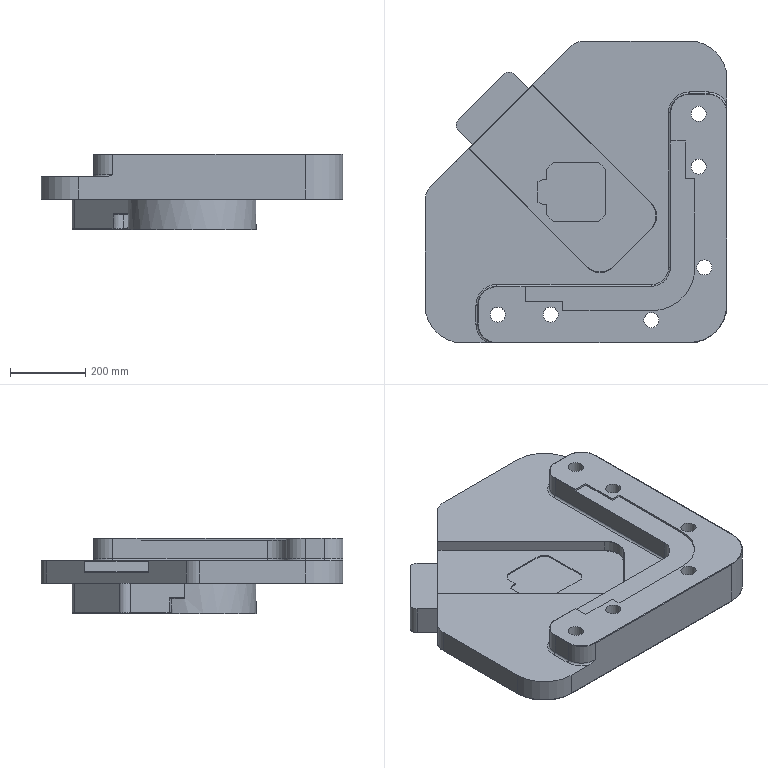Component | NX | TRANSITION_ACTUATOR_FLANGE | 2 solids | 222 faces | volume 46455477 mm3 | cylinder 105 | plane 91 | torus 26 | commonest cylinder face diameters 2 x21 12 x14 25 x12 40 x10 100 x9 23 x8 4 x6 65 x6